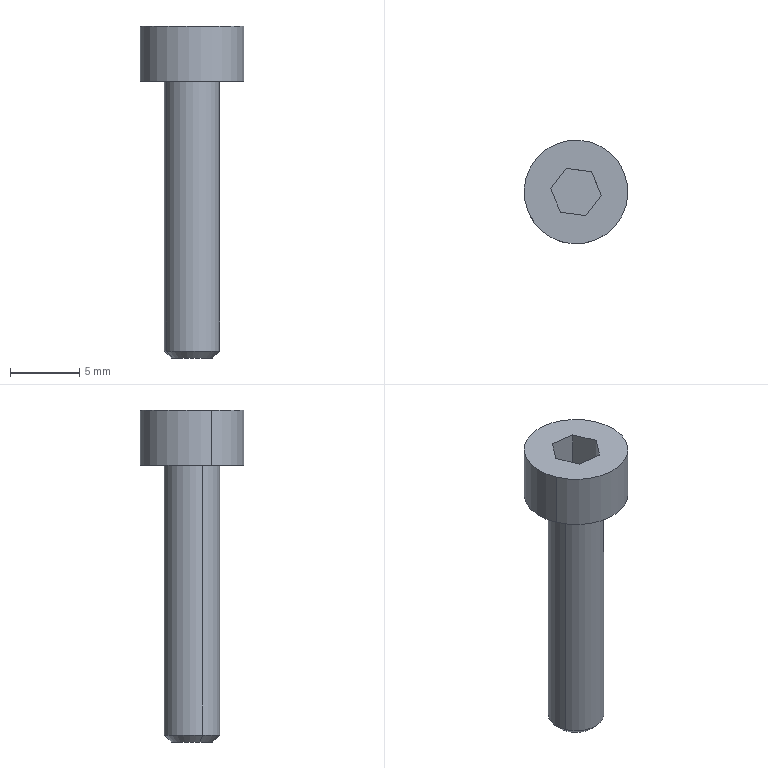Component | SolidWorks | M4x20HexSocketCapScrew-1 | 1 solid | 16 faces | box 7.5 x 7.5 x 24 mm | volume 400 mm3 | plane 10 | cylinder 4 | cone 2 | commonest cylinder face diameters 4 x2 7.5 x2 | material #45
STEP:
#1=COLOUR_RGB('',0.7922,0.8196,0.9333);
#2=FILL_AREA_STYLE_COLOUR('',#1);
#3=FILL_AREA_STYLE('',(#2));
#4=SURFACE_STYLE_FILL_AREA(#3);
#5=SURFACE_SIDE_STYLE('',(#4));
#6=SURFACE_STYLE_USAGE(.BOTH.,#5);
#7=PRESENTATION_STYLE_ASSIGNMENT((#6));
#8=CARTESIAN_POINT('',(3.97,-2.523,-0.09843));
#9=VERTEX_POINT('',#8);
#10=CARTESIAN_POINT('',(4.079,-2.477,-0.09843));
#11=VERTEX_POINT('',#10);
#12=CARTESIAN_POINT('',(4.024,-2.5,-0.09843));
#13=DIRECTION('',(0.,0.,-1.));
#14=DIRECTION('',(-0.9237,-0.383,0.));
#15=AXIS2_PLACEMENT_3D('',#12,#13,#14);
#16=CIRCLE('',#15,0.05906);
#17=EDGE_CURVE('',#9,#11,#16,.T.);
#18=ORIENTED_EDGE('',*,*,#17,.F.);
#19=CARTESIAN_POINT('',(3.951,-2.53,-0.07874));
#20=VERTEX_POINT('',#19);
#21=CARTESIAN_POINT('',(3.951,-2.53,-0.07874));
#22=DIRECTION('',(-0.6532,-0.2709,0.7071));
#23=VECTOR('',#22,39.37);
#24=LINE('',#21,#23);
#25=EDGE_CURVE('',#9,#20,#24,.T.);
#26=ORIENTED_EDGE('',*,*,#25,.T.);
#27=CARTESIAN_POINT('',(4.097,-2.47,-0.07874));
#28=VERTEX_POINT('',#27);
#29=CARTESIAN_POINT('',(4.024,-2.5,-0.07874));
#30=DIRECTION('',(0.,0.,-1.));
#31=DIRECTION('',(-0.9237,-0.383,0.));
#32=AXIS2_PLACEMENT_3D('',#29,#30,#31);
#33=CIRCLE('',#32,0.07874);
#34=EDGE_CURVE('',#20,#28,#33,.T.);
#35=ORIENTED_EDGE('',*,*,#34,.T.);
#36=CARTESIAN_POINT('',(4.097,-2.47,-0.07874));
#37=DIRECTION('',(0.6532,0.2709,0.7071));
#38=VECTOR('',#37,39.37);
#39=LINE('',#36,#38);
#40=EDGE_CURVE('',#11,#28,#39,.T.);
#41=ORIENTED_EDGE('',*,*,#40,.F.);
#42=EDGE_LOOP('',(#18,#26,#35,#41));
#43=FACE_OUTER_BOUND('',#42,.T.);
#44=CARTESIAN_POINT('',(4.024,-2.5,-0.07874));
#45=DIRECTION('',(0.,-0.,1.));
#46=DIRECTION('',(0.9237,0.383,0.));
#47=AXIS2_PLACEMENT_3D('',#44,#45,#46);
#48=CONICAL_SURFACE('',#47,0.07874,0.7854);
#49=ADVANCED_FACE('',(#43),#48,.T.);
#50=CARTESIAN_POINT('',(3.951,-2.53,0.689));
#51=VERTEX_POINT('',#50);
#52=CARTESIAN_POINT('',(4.097,-2.47,0.689));
#53=VERTEX_POINT('',#52);
#54=CARTESIAN_POINT('',(4.024,-2.5,0.689));
#55=DIRECTION('',(0.,0.,-1.));
#56=DIRECTION('',(-0.9237,-0.383,0.));
#57=AXIS2_PLACEMENT_3D('',#54,#55,#56);
#58=CIRCLE('',#57,0.07874);
#59=EDGE_CURVE('',#51,#53,#58,.T.);
#60=ORIENTED_EDGE('',*,*,#59,.T.);
#61=CARTESIAN_POINT('',(4.097,-2.47,-0.09843));
#62=DIRECTION('',(0.,0.,-1.));
#63=VECTOR('',#62,39.37);
#64=LINE('',#61,#63);
#65=EDGE_CURVE('',#53,#28,#64,.T.);
#66=ORIENTED_EDGE('',*,*,#65,.T.);
#67=ORIENTED_EDGE('',*,*,#34,.F.);
#68=CARTESIAN_POINT('',(3.951,-2.53,-0.09843));
#69=DIRECTION('',(0.,0.,-1.));
#70=VECTOR('',#69,39.37);
#71=LINE('',#68,#70);
#72=EDGE_CURVE('',#51,#20,#71,.T.);
#73=ORIENTED_EDGE('',*,*,#72,.F.);
#74=EDGE_LOOP('',(#60,#66,#67,#73));
#75=FACE_OUTER_BOUND('',#74,.T.);
#76=CARTESIAN_POINT('',(4.024,-2.5,-0.09843));
#77=DIRECTION('',(0.,0.,-1.));
#78=DIRECTION('',(-0.9237,-0.383,0.));
#79=AXIS2_PLACEMENT_3D('',#76,#77,#78);
#80=CYLINDRICAL_SURFACE('',#79,0.07874);
#81=ADVANCED_FACE('',(#75),#80,.T.);
#82=CARTESIAN_POINT('',(3.888,-2.557,0.8465));
#83=VERTEX_POINT('',#82);
#84=CARTESIAN_POINT('',(4.161,-2.443,0.8465));
#85=VERTEX_POINT('',#84);
#86=CARTESIAN_POINT('',(4.024,-2.5,0.8465));
#87=DIRECTION('',(0.,0.,-1.));
#88=DIRECTION('',(-0.9237,-0.383,0.));
#89=AXIS2_PLACEMENT_3D('',#86,#87,#88);
#90=CIRCLE('',#89,0.1476);
#91=EDGE_CURVE('',#83,#85,#90,.T.);
#92=ORIENTED_EDGE('',*,*,#91,.T.);
#93=CARTESIAN_POINT('',(4.161,-2.443,0.689));
#94=VERTEX_POINT('',#93);
#95=CARTESIAN_POINT('',(4.161,-2.443,-0.09843));
#96=DIRECTION('',(0.,0.,-1.));
#97=VECTOR('',#96,39.37);
#98=LINE('',#95,#97);
#99=EDGE_CURVE('',#85,#94,#98,.T.);
#100=ORIENTED_EDGE('',*,*,#99,.T.);
#101=CARTESIAN_POINT('',(3.888,-2.557,0.689));
#102=VERTEX_POINT('',#101);
#103=CARTESIAN_POINT('',(4.024,-2.5,0.689));
#104=DIRECTION('',(0.,0.,-1.));
#105=DIRECTION('',(-0.9237,-0.383,0.));
#106=AXIS2_PLACEMENT_3D('',#103,#104,#105);
#107=CIRCLE('',#106,0.1476);
#108=EDGE_CURVE('',#102,#94,#107,.T.);
#109=ORIENTED_EDGE('',*,*,#108,.F.);
#110=CARTESIAN_POINT('',(3.888,-2.557,-0.09843));
#111=DIRECTION('',(0.,0.,-1.));
#112=VECTOR('',#111,39.37);
#113=LINE('',#110,#112);
#114=EDGE_CURVE('',#83,#102,#113,.T.);
#115=ORIENTED_EDGE('',*,*,#114,.F.);
#116=EDGE_LOOP('',(#92,#100,#109,#115));
#117=FACE_OUTER_BOUND('',#116,.T.);
#118=CARTESIAN_POINT('',(4.024,-2.5,-0.09843));
#119=DIRECTION('',(0.,0.,-1.));
#120=DIRECTION('',(-0.9237,-0.383,0.));
#121=AXIS2_PLACEMENT_3D('',#118,#119,#120);
#122=CYLINDRICAL_SURFACE('',#121,0.1476);
#123=ADVANCED_FACE('',(#117),#122,.T.);
#124=CARTESIAN_POINT('',(3.996,-2.433,0.8465));
#125=VERTEX_POINT('',#124);
#126=CARTESIAN_POINT('',(3.952,-2.491,0.8465));
#127=VERTEX_POINT('',#126);
#128=CARTESIAN_POINT('',(3.996,-2.433,0.8465));
#129=DIRECTION('',(-0.6084,-0.7936,-0.));
#130=VECTOR('',#129,39.37);
#131=LINE('',#128,#130);
#132=EDGE_CURVE('',#125,#127,#131,.T.);
#133=ORIENTED_EDGE('',*,*,#132,.F.);
#134=CARTESIAN_POINT('',(4.068,-2.442,0.8465));
#135=VERTEX_POINT('',#134);
#136=CARTESIAN_POINT('',(4.068,-2.442,0.8465));
#137=DIRECTION('',(-0.9915,0.1301,-0.));
#138=VECTOR('',#137,39.37);
#139=LINE('',#136,#138);
#140=EDGE_CURVE('',#135,#125,#139,.T.);
#141=ORIENTED_EDGE('',*,*,#140,.F.);
#142=CARTESIAN_POINT('',(4.096,-2.509,0.8465));
#143=VERTEX_POINT('',#142);
#144=CARTESIAN_POINT('',(4.096,-2.509,0.8465));
#145=DIRECTION('',(-0.383,0.9237,0.));
#146=VECTOR('',#145,39.37);
#147=LINE('',#144,#146);
#148=EDGE_CURVE('',#143,#135,#147,.T.);
#149=ORIENTED_EDGE('',*,*,#148,.F.);
#150=CARTESIAN_POINT('',(4.052,-2.567,0.8465));
#151=VERTEX_POINT('',#150);
#152=CARTESIAN_POINT('',(4.052,-2.567,0.8465));
#153=DIRECTION('',(0.6084,0.7936,0.));
#154=VECTOR('',#153,39.37);
#155=LINE('',#152,#154);
#156=EDGE_CURVE('',#151,#143,#155,.T.);
#157=ORIENTED_EDGE('',*,*,#156,.F.);
#158=CARTESIAN_POINT('',(3.98,-2.558,0.8465));
#159=VERTEX_POINT('',#158);
#160=CARTESIAN_POINT('',(3.98,-2.558,0.8465));
#161=DIRECTION('',(0.9915,-0.1301,0.));
#162=VECTOR('',#161,39.37);
#163=LINE('',#160,#162);
#164=EDGE_CURVE('',#159,#151,#163,.T.);
#165=ORIENTED_EDGE('',*,*,#164,.F.);
#166=CARTESIAN_POINT('',(3.952,-2.491,0.8465));
#167=DIRECTION('',(0.383,-0.9237,-0.));
#168=VECTOR('',#167,39.37);
#169=LINE('',#166,#168);
#170=EDGE_CURVE('',#127,#159,#169,.T.);
#171=ORIENTED_EDGE('',*,*,#170,.F.);
#172=EDGE_LOOP('',(#133,#141,#149,#157,#165,#171));
#173=FACE_BOUND('',#172,.T.);
#174=ORIENTED_EDGE('',*,*,#91,.F.);
#175=CARTESIAN_POINT('',(4.024,-2.5,0.8465));
#176=DIRECTION('',(0.,0.,-1.));
#177=DIRECTION('',(-0.9237,-0.383,0.));
#178=AXIS2_PLACEMENT_3D('',#175,#176,#177);
#179=CIRCLE('',#178,0.1476);
#180=EDGE_CURVE('',#85,#83,#179,.T.);
#181=ORIENTED_EDGE('',*,*,#180,.F.);
#182=EDGE_LOOP('',(#174,#181));
#183=FACE_OUTER_BOUND('',#182,.T.);
#184=CARTESIAN_POINT('',(4.024,-2.5,0.8465));
#185=DIRECTION('',(0.,0.,-1.));
#186=DIRECTION('',(-0.9237,-0.383,-0.));
#187=AXIS2_PLACEMENT_3D('',#184,#185,#186);
#188=PLANE('',#187);
#189=ADVANCED_FACE('',(#173,#183),#188,.F.);
#190=ORIENTED_EDGE('',*,*,#99,.F.);
#191=ORIENTED_EDGE('',*,*,#180,.T.);
#192=ORIENTED_EDGE('',*,*,#114,.T.);
#193=CARTESIAN_POINT('',(4.024,-2.5,0.689));
#194=DIRECTION('',(0.,0.,-1.));
#195=DIRECTION('',(-0.9237,-0.383,0.));
#196=AXIS2_PLACEMENT_3D('',#193,#194,#195);
#197=CIRCLE('',#196,0.1476);
#198=EDGE_CURVE('',#94,#102,#197,.T.);
#199=ORIENTED_EDGE('',*,*,#198,.F.);
#200=EDGE_LOOP('',(#190,#191,#192,#199));
#201=FACE_OUTER_BOUND('',#200,.T.);
#202=CARTESIAN_POINT('',(4.024,-2.5,-0.09843));
#203=DIRECTION('',(0.,0.,-1.));
#204=DIRECTION('',(-0.9237,-0.383,0.));
#205=AXIS2_PLACEMENT_3D('',#202,#203,#204);
#206=CYLINDRICAL_SURFACE('',#205,0.1476);
#207=ADVANCED_FACE('',(#201),#206,.T.);
#208=ORIENTED_EDGE('',*,*,#59,.F.);
#209=CARTESIAN_POINT('',(4.024,-2.5,0.689));
#210=DIRECTION('',(0.,0.,-1.));
#211=DIRECTION('',(-0.9237,-0.383,0.));
#212=AXIS2_PLACEMENT_3D('',#209,#210,#211);
#213=CIRCLE('',#212,0.07874);
#214=EDGE_CURVE('',#53,#51,#213,.T.);
#215=ORIENTED_EDGE('',*,*,#214,.F.);
#216=EDGE_LOOP('',(#208,#215));
#217=FACE_BOUND('',#216,.T.);
#218=ORIENTED_EDGE('',*,*,#108,.T.);
#219=ORIENTED_EDGE('',*,*,#198,.T.);
#220=EDGE_LOOP('',(#218,#219));
#221=FACE_OUTER_BOUND('',#220,.T.);
#222=CARTESIAN_POINT('',(4.161,-2.443,0.689));
#223=DIRECTION('',(-0.,-0.,1.));
#224=DIRECTION('',(0.9237,0.383,0.));
#225=AXIS2_PLACEMENT_3D('',#222,#223,#224);
#226=PLANE('',#225);
#227=ADVANCED_FACE('',(#217,#221),#226,.F.);
#228=ORIENTED_EDGE('',*,*,#65,.F.);
#229=ORIENTED_EDGE('',*,*,#214,.T.);
#230=ORIENTED_EDGE('',*,*,#72,.T.);
#231=CARTESIAN_POINT('',(4.024,-2.5,-0.07874));
#232=DIRECTION('',(0.,0.,-1.));
#233=DIRECTION('',(-0.9237,-0.383,0.));
#234=AXIS2_PLACEMENT_3D('',#231,#232,#233);
#235=CIRCLE('',#234,0.07874);
#236=EDGE_CURVE('',#28,#20,#235,.T.);
#237=ORIENTED_EDGE('',*,*,#236,.F.);
#238=EDGE_LOOP('',(#228,#229,#230,#237));
#239=FACE_OUTER_BOUND('',#238,.T.);
#240=CARTESIAN_POINT('',(4.024,-2.5,-0.09843));
#241=DIRECTION('',(0.,0.,-1.));
#242=DIRECTION('',(-0.9237,-0.383,0.));
#243=AXIS2_PLACEMENT_3D('',#240,#241,#242);
#244=CYLINDRICAL_SURFACE('',#243,0.07874);
#245=ADVANCED_FACE('',(#239),#244,.T.);
#246=ORIENTED_EDGE('',*,*,#25,.F.);
#247=CARTESIAN_POINT('',(4.024,-2.5,-0.09843));
#248=DIRECTION('',(0.,0.,-1.));
#249=DIRECTION('',(-0.9237,-0.383,0.));
#250=AXIS2_PLACEMENT_3D('',#247,#248,#249);
#251=CIRCLE('',#250,0.05906);
#252=EDGE_CURVE('',#11,#9,#251,.T.);
#253=ORIENTED_EDGE('',*,*,#252,.F.);
#254=ORIENTED_EDGE('',*,*,#40,.T.);
#255=ORIENTED_EDGE('',*,*,#236,.T.);
#256=EDGE_LOOP('',(#246,#253,#254,#255));
#257=FACE_OUTER_BOUND('',#256,.T.);
#258=CARTESIAN_POINT('',(4.024,-2.5,-0.07874));
#259=DIRECTION('',(0.,-0.,1.));
#260=DIRECTION('',(0.9237,0.383,0.));
#261=AXIS2_PLACEMENT_3D('',#258,#259,#260);
#262=CONICAL_SURFACE('',#261,0.07874,0.7854);
#263=ADVANCED_FACE('',(#257),#262,.T.);
#264=ORIENTED_EDGE('',*,*,#252,.T.);
#265=ORIENTED_EDGE('',*,*,#17,.T.);
#266=EDGE_LOOP('',(#264,#265));
#267=FACE_OUTER_BOUND('',#266,.T.);
#268=CARTESIAN_POINT('',(4.079,-2.477,-0.09843));
#269=DIRECTION('',(-0.,-0.,1.));
#270=DIRECTION('',(0.9237,0.383,0.));
#271=AXIS2_PLACEMENT_3D('',#268,#269,#270);
#272=PLANE('',#271);
#273=ADVANCED_FACE('',(#267),#272,.F.);
#274=ORIENTED_EDGE('',*,*,#140,.T.);
#275=CARTESIAN_POINT('',(3.996,-2.433,0.7283));
#276=VERTEX_POINT('',#275);
#277=CARTESIAN_POINT('',(3.996,-2.433,0.7283));
#278=DIRECTION('',(0.,-0.,1.));
#279=VECTOR('',#278,39.37);
#280=LINE('',#277,#279);
#281=EDGE_CURVE('',#276,#125,#280,.T.);
#282=ORIENTED_EDGE('',*,*,#281,.F.);
#283=CARTESIAN_POINT('',(4.068,-2.442,0.7283));
#284=VERTEX_POINT('',#283);
#285=CARTESIAN_POINT('',(4.068,-2.442,0.7283));
#286=DIRECTION('',(-0.9915,0.1301,-0.));
#287=VECTOR('',#286,39.37);
#288=LINE('',#285,#287);
#289=EDGE_CURVE('',#284,#276,#288,.T.);
#290=ORIENTED_EDGE('',*,*,#289,.F.);
#291=CARTESIAN_POINT('',(4.068,-2.442,0.7283));
#292=DIRECTION('',(0.,-0.,1.));
#293=VECTOR('',#292,39.37);
#294=LINE('',#291,#293);
#295=EDGE_CURVE('',#284,#135,#294,.T.);
#296=ORIENTED_EDGE('',*,*,#295,.T.);
#297=EDGE_LOOP('',(#274,#282,#290,#296));
#298=FACE_OUTER_BOUND('',#297,.T.);
#299=CARTESIAN_POINT('',(4.068,-2.442,0.7283));
#300=DIRECTION('',(0.1301,0.9915,0.));
#301=DIRECTION('',(0.9915,-0.1301,0.));
#302=AXIS2_PLACEMENT_3D('',#299,#300,#301);
#303=PLANE('',#302);
#304=ADVANCED_FACE('',(#298),#303,.F.);
#305=ORIENTED_EDGE('',*,*,#148,.T.);
#306=ORIENTED_EDGE('',*,*,#295,.F.);
#307=CARTESIAN_POINT('',(4.096,-2.509,0.7283));
#308=VERTEX_POINT('',#307);
#309=CARTESIAN_POINT('',(4.096,-2.509,0.7283));
#310=DIRECTION('',(-0.383,0.9237,0.));
#311=VECTOR('',#310,39.37);
#312=LINE('',#309,#311);
#313=EDGE_CURVE('',#308,#284,#312,.T.);
#314=ORIENTED_EDGE('',*,*,#313,.F.);
#315=CARTESIAN_POINT('',(4.096,-2.509,0.7283));
#316=DIRECTION('',(0.,-0.,1.));
#317=VECTOR('',#316,39.37);
#318=LINE('',#315,#317);
#319=EDGE_CURVE('',#308,#143,#318,.T.);
#320=ORIENTED_EDGE('',*,*,#319,.T.);
#321=EDGE_LOOP('',(#305,#306,#314,#320));
#322=FACE_OUTER_BOUND('',#321,.T.);
#323=CARTESIAN_POINT('',(4.096,-2.509,0.7283));
#324=DIRECTION('',(0.9237,0.383,0.));
#325=DIRECTION('',(0.383,-0.9237,-0.));
#326=AXIS2_PLACEMENT_3D('',#323,#324,#325);
#327=PLANE('',#326);
#328=ADVANCED_FACE('',(#322),#327,.F.);
#329=ORIENTED_EDGE('',*,*,#156,.T.);
#330=ORIENTED_EDGE('',*,*,#319,.F.);
#331=CARTESIAN_POINT('',(4.052,-2.567,0.7283));
#332=VERTEX_POINT('',#331);
#333=CARTESIAN_POINT('',(4.052,-2.567,0.7283));
#334=DIRECTION('',(0.6084,0.7936,0.));
#335=VECTOR('',#334,39.37);
#336=LINE('',#333,#335);
#337=EDGE_CURVE('',#332,#308,#336,.T.);
#338=ORIENTED_EDGE('',*,*,#337,.F.);
#339=CARTESIAN_POINT('',(4.052,-2.567,0.7283));
#340=DIRECTION('',(0.,-0.,1.));
#341=VECTOR('',#340,39.37);
#342=LINE('',#339,#341);
#343=EDGE_CURVE('',#332,#151,#342,.T.);
#344=ORIENTED_EDGE('',*,*,#343,.T.);
#345=EDGE_LOOP('',(#329,#330,#338,#344));
#346=FACE_OUTER_BOUND('',#345,.T.);
#347=CARTESIAN_POINT('',(4.052,-2.567,0.7283));
#348=DIRECTION('',(0.7936,-0.6084,-0.));
#349=DIRECTION('',(-0.6084,-0.7936,-0.));
#350=AXIS2_PLACEMENT_3D('',#347,#348,#349);
#351=PLANE('',#350);
#352=ADVANCED_FACE('',(#346),#351,.F.);
#353=ORIENTED_EDGE('',*,*,#164,.T.);
#354=ORIENTED_EDGE('',*,*,#343,.F.);
#355=CARTESIAN_POINT('',(3.98,-2.558,0.7283));
#356=VERTEX_POINT('',#355);
#357=CARTESIAN_POINT('',(3.98,-2.558,0.7283));
#358=DIRECTION('',(0.9915,-0.1301,0.));
#359=VECTOR('',#358,39.37);
#360=LINE('',#357,#359);
#361=EDGE_CURVE('',#356,#332,#360,.T.);
#362=ORIENTED_EDGE('',*,*,#361,.F.);
#363=CARTESIAN_POINT('',(3.98,-2.558,0.7283));
#364=DIRECTION('',(0.,-0.,1.));
#365=VECTOR('',#364,39.37);
#366=LINE('',#363,#365);
#367=EDGE_CURVE('',#356,#159,#366,.T.);
#368=ORIENTED_EDGE('',*,*,#367,.T.);
#369=EDGE_LOOP('',(#353,#354,#362,#368));
#370=FACE_OUTER_BOUND('',#369,.T.);
#371=CARTESIAN_POINT('',(3.98,-2.558,0.7283));
#372=DIRECTION('',(-0.1301,-0.9915,-0.));
#373=DIRECTION('',(-0.9915,0.1301,-0.));
#374=AXIS2_PLACEMENT_3D('',#371,#372,#373);
#375=PLANE('',#374);
#376=ADVANCED_FACE('',(#370),#375,.F.);
#377=ORIENTED_EDGE('',*,*,#170,.T.);
#378=ORIENTED_EDGE('',*,*,#367,.F.);
#379=CARTESIAN_POINT('',(3.952,-2.491,0.7283));
#380=VERTEX_POINT('',#379);
#381=CARTESIAN_POINT('',(3.952,-2.491,0.7283));
#382=DIRECTION('',(0.383,-0.9237,-0.));
#383=VECTOR('',#382,39.37);
#384=LINE('',#381,#383);
#385=EDGE_CURVE('',#380,#356,#384,.T.);
#386=ORIENTED_EDGE('',*,*,#385,.F.);
#387=CARTESIAN_POINT('',(3.952,-2.491,0.7283));
#388=DIRECTION('',(0.,-0.,1.));
#389=VECTOR('',#388,39.37);
#390=LINE('',#387,#389);
#391=EDGE_CURVE('',#380,#127,#390,.T.);
#392=ORIENTED_EDGE('',*,*,#391,.T.);
#393=EDGE_LOOP('',(#377,#378,#386,#392));
#394=FACE_OUTER_BOUND('',#393,.T.);
#395=CARTESIAN_POINT('',(3.952,-2.491,0.7283));
#396=DIRECTION('',(-0.9237,-0.383,-0.));
#397=DIRECTION('',(0.,-0.,1.));
#398=AXIS2_PLACEMENT_3D('',#395,#396,#397);
#399=PLANE('',#398);
#400=ADVANCED_FACE('',(#394),#399,.F.);
#401=ORIENTED_EDGE('',*,*,#132,.T.);
#402=ORIENTED_EDGE('',*,*,#391,.F.);
#403=CARTESIAN_POINT('',(3.996,-2.433,0.7283));
#404=DIRECTION('',(-0.6084,-0.7936,-0.));
#405=VECTOR('',#404,39.37);
#406=LINE('',#403,#405);
#407=EDGE_CURVE('',#276,#380,#406,.T.);
#408=ORIENTED_EDGE('',*,*,#407,.F.);
#409=ORIENTED_EDGE('',*,*,#281,.T.);
#410=EDGE_LOOP('',(#401,#402,#408,#409));
#411=FACE_OUTER_BOUND('',#410,.T.);
#412=CARTESIAN_POINT('',(3.996,-2.433,0.7283));
#413=DIRECTION('',(-0.7936,0.6084,0.));
#414=DIRECTION('',(0.6084,0.7936,0.));
#415=AXIS2_PLACEMENT_3D('',#412,#413,#414);
#416=PLANE('',#415);
#417=ADVANCED_FACE('',(#411),#416,.F.);
#418=ORIENTED_EDGE('',*,*,#289,.T.);
#419=ORIENTED_EDGE('',*,*,#407,.T.);
#420=ORIENTED_EDGE('',*,*,#385,.T.);
#421=ORIENTED_EDGE('',*,*,#361,.T.);
#422=ORIENTED_EDGE('',*,*,#337,.T.);
#423=ORIENTED_EDGE('',*,*,#313,.T.);
#424=EDGE_LOOP('',(#418,#419,#420,#421,#422,#423));
#425=FACE_OUTER_BOUND('',#424,.T.);
#426=CARTESIAN_POINT('',(4.024,-2.5,0.7283));
#427=DIRECTION('',(-0.,-0.,1.));
#428=DIRECTION('',(0.9237,0.383,0.));
#429=AXIS2_PLACEMENT_3D('',#426,#427,#428);
#430=PLANE('',#429);
#431=ADVANCED_FACE('',(#425),#430,.T.);
#432=CLOSED_SHELL('',(#49,#81,#123,#189,#207,#227,#245,#263,#273,#304,#328,#352,#376,#400,#417,#431));
#433=MANIFOLD_SOLID_BREP('',#432);
#434=STYLED_ITEM('',(#7),#433);
#435=(LENGTH_UNIT()NAMED_UNIT(*)SI_UNIT($,.METRE.));
#436=LENGTH_MEASURE_WITH_UNIT(LENGTH_MEASURE(0.0254),#435);
#437=DIMENSIONAL_EXPONENTS(1.,0.,0.,0.,0.,0.,0.);
#438=(CONVERSION_BASED_UNIT('',#436)LENGTH_UNIT()NAMED_UNIT(#437));
#439=UNCERTAINTY_MEASURE_WITH_UNIT(LENGTH_MEASURE(0.00001),#438,'','');
#440=(NAMED_UNIT(*)PLANE_ANGLE_UNIT()SI_UNIT($,.RADIAN.));
#441=(NAMED_UNIT(*)SI_UNIT($,.STERADIAN.)SOLID_ANGLE_UNIT());
#442=(GEOMETRIC_REPRESENTATION_CONTEXT(3)GLOBAL_UNCERTAINTY_ASSIGNED_CONTEXT((#439))GLOBAL_UNIT_ASSIGNED_CONTEXT((#438,#440,#441))REPRESENTATION_CONTEXT('',''));
#443=MECHANICAL_DESIGN_GEOMETRIC_PRESENTATION_REPRESENTATION('',(#434),#442);
#444=PRESENTATION_LAYER_ASSIGNMENT('','',(#434));
#445=CARTESIAN_POINT('',(0.,0.,0.));
#446=DIRECTION('',(0.,0.,1.));
#447=DIRECTION('',(1.,0.,0.));
#448=AXIS2_PLACEMENT_3D('',#445,#446,#447);
#449=(LENGTH_UNIT()NAMED_UNIT(*)SI_UNIT($,.METRE.));
#450=LENGTH_MEASURE_WITH_UNIT(LENGTH_MEASURE(0.0254),#449);
#451=DIMENSIONAL_EXPONENTS(1.,0.,0.,0.,0.,0.,0.);
#452=(CONVERSION_BASED_UNIT('',#450)LENGTH_UNIT()NAMED_UNIT(#451));
#453=UNCERTAINTY_MEASURE_WITH_UNIT(LENGTH_MEASURE(0.00001),#452,'','');
#454=(NAMED_UNIT(*)PLANE_ANGLE_UNIT()SI_UNIT($,.RADIAN.));
#455=(NAMED_UNIT(*)SI_UNIT($,.STERADIAN.)SOLID_ANGLE_UNIT());
#456=(GEOMETRIC_REPRESENTATION_CONTEXT(3)GLOBAL_UNCERTAINTY_ASSIGNED_CONTEXT((#453))GLOBAL_UNIT_ASSIGNED_CONTEXT((#452,#454,#455))REPRESENTATION_CONTEXT('',''));
#457=ADVANCED_BREP_SHAPE_REPRESENTATION('',(#433,#448),#456);